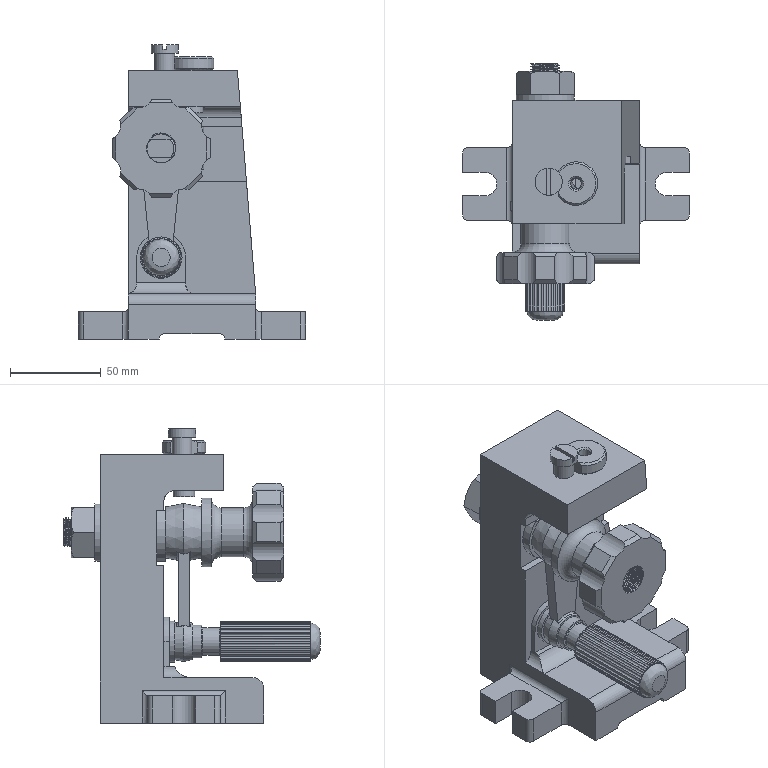Assembly | NX | mm | 11 component files | 11 solids | 437 faces | box 125 x 141 x 162 mm | volume 598113 mm3 | cylinder 187 | plane 153 | spline 64 | cone 23 | torus 10 | commonest cylinder face diameters 16 x51 14 x27 21.6 x25 1.6 x25 6 x14 12 x9 20 x5 13 x4
Bill of materials:
unnamed part 1 | 1 |  | Stepped turned shaft/stud with external threads on both ends, a larger plain cylindrical body, and a raised collar that looks faceted.
unnamed part 2 | 1 |  | Block-style bracket shaped like a C or L, with an overhanging top arm, an upright wall with a sloped back, and a base plate with two side ears that have open U-slots.
unnamed part 3 | 1 |  | Plain flat washer: a thin ring of constant thickness with a central round hole.
unnamed part 4 | 1 |  | Flanged cylindrical bushing with a through bore and a chamfer on the end away from the flange.
unnamed part 5 | 1 |  | Cylindrical sleeve/spacer with a through bore and a larger-diameter counterbore step at one end.
unnamed part 6 | 1 |  | Hexagonal nut with an internally threaded through hole and chamfered corners.
unnamed part 7 | 1 |  | Stepped pin or plunger with a domed end, a long section with lengthwise flutes or serrations, a collar, and a smaller plain pin at the other end.
unnamed part 8 | 1 |  | Lever or link arm with a large split clamp eye at one end, a tapered web, and a smaller round eye at the other end.
unnamed part 9 | 1 |  | Spool-shaped knob with a scalloped, lobed grip end, a waisted neck with fillets, a thin end flange, and a central bore.
unnamed part 10 | 1 |  | Slotted shoulder screw: a cylindrical head with a straight drive slot, a plain larger-diameter shoulder, and a smaller threaded tip with an undercut.
unnamed part 11 | 1 |  | Headed pin or bushing with a chamfered head that has one flat or cut-off side, a short step under the head, a long plain cylindrical shank, and a central hole in the head.
Mates:
1. fix | Stand 1 component
2. touch align | Locating_Bush 1 face | Stand 1 face
3. touch align | Locating_Bush 1 face | Stand 1 face
4. touch align | Locating_Peg 1 face | Stand 1 face
5. touch align | Locating_Peg 1 face | Stand 1 face
6. touch align | Washer 1 face | Locating_Peg 1 face
7. touch align | Washer 1 face | Stand 1 face
8. touch align | Nut_M16 1 face | Locating_Peg 1 face
9. touch align | Nut_M16 1 face | Washer 1 face
10. touch align | Liner_Bush 1 face | Stand 1 face
11. touch align | Liner_Bush 1 face | Stand 1 face
12. touch align | Guide_Bush_1 1 face | Liner_Bush 1 face
13. touch align | Guide_Bush_1 1 face | Stand 1 face
14. touch align | Locking_Screw 1 face | Stand 1 face
15. touch align | Locking_Screw 1 face | Stand 1 face
16. touch align | Lever 1 face | Locating_Peg 1 face
17. touch align | Lever 1 face | Locating_Peg 1 face
18. touch align | Locating_Plug 1 face | Lever 1 face
19. touch align | Locating_Plug 1 face | Lever 1 face
20. touch align | Hand_Nut 1 face | Lever 1 face
21. touch align | Hand_Nut 1 face | Lever 1 face